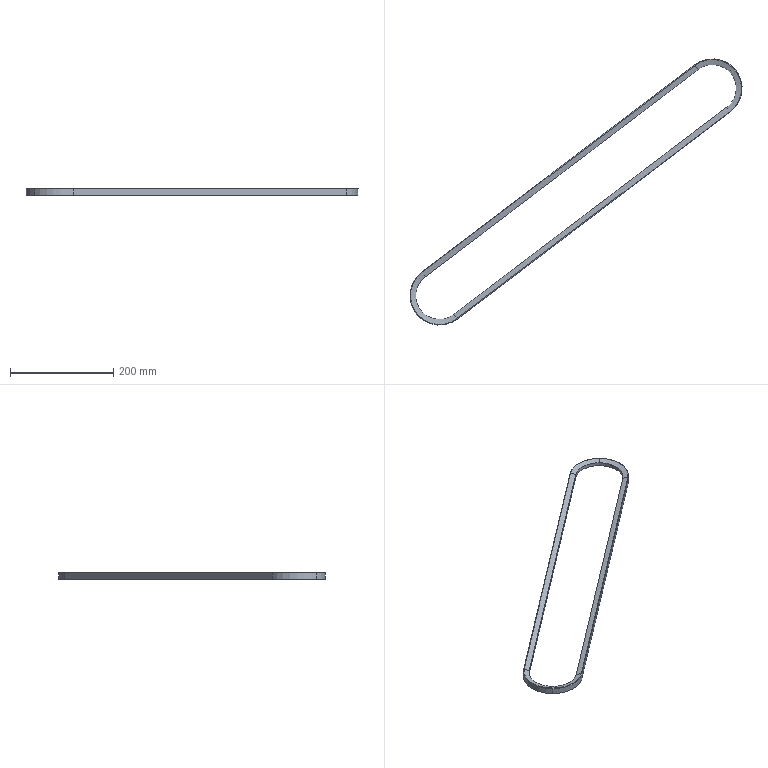Component | SolidWorks | Belt-1 | 1 solid | 30 faces | box 643.7 x 516.05 x 13.2 mm | volume 188359 mm3 | cone 12 | plane 12 | cylinder 6 | commonest cylinder face diameters 114 x3 92 x3
STEP:
#1=COLOUR_RGB('',0.7922,0.8196,0.9333);
#2=FILL_AREA_STYLE_COLOUR('',#1);
#3=FILL_AREA_STYLE('',(#2));
#4=SURFACE_STYLE_FILL_AREA(#3);
#5=SURFACE_SIDE_STYLE('',(#4));
#6=SURFACE_STYLE_USAGE(.BOTH.,#5);
#7=PRESENTATION_STYLE_ASSIGNMENT((#6));
#8=CARTESIAN_POINT('',(-11.222,-8.795,-9.154));
#9=VERTEX_POINT('',#8);
#10=CARTESIAN_POINT('',(-14.155,-8.605,-9.154));
#11=VERTEX_POINT('',#10);
#12=CARTESIAN_POINT('',(-12.579,-7.008,-9.154));
#13=DIRECTION('',(0.,0.,-1.));
#14=DIRECTION('',(-0.7024,-0.7117,0.));
#15=AXIS2_PLACEMENT_3D('',#12,#13,#14);
#16=CIRCLE('',#15,2.244);
#17=EDGE_CURVE('',#9,#11,#16,.T.);
#18=ORIENTED_EDGE('',*,*,#17,.T.);
#19=CARTESIAN_POINT('',(-14.155,-8.605,-9.618));
#20=VERTEX_POINT('',#19);
#21=CARTESIAN_POINT('',(-14.155,-8.605,-9.386));
#22=DIRECTION('',(0.,0.,-1.));
#23=VECTOR('',#22,39.37);
#24=LINE('',#21,#23);
#25=EDGE_CURVE('',#11,#20,#24,.T.);
#26=ORIENTED_EDGE('',*,*,#25,.T.);
#27=CARTESIAN_POINT('',(-11.222,-8.795,-9.618));
#28=VERTEX_POINT('',#27);
#29=CARTESIAN_POINT('',(-12.579,-7.008,-9.618));
#30=DIRECTION('',(0.,0.,1.));
#31=DIRECTION('',(-0.7024,-0.7117,0.));
#32=AXIS2_PLACEMENT_3D('',#29,#30,#31);
#33=CIRCLE('',#32,2.244);
#34=EDGE_CURVE('',#20,#28,#33,.T.);
#35=ORIENTED_EDGE('',*,*,#34,.T.);
#36=CARTESIAN_POINT('',(-11.222,-8.795,-9.386));
#37=DIRECTION('',(0.,0.,1.));
#38=VECTOR('',#37,39.37);
#39=LINE('',#36,#38);
#40=EDGE_CURVE('',#28,#9,#39,.T.);
#41=ORIENTED_EDGE('',*,*,#40,.T.);
#42=EDGE_LOOP('',(#18,#26,#35,#41));
#43=FACE_OUTER_BOUND('',#42,.T.);
#44=CARTESIAN_POINT('',(-12.579,-7.008,-9.386));
#45=DIRECTION('',(0.,0.,-1.));
#46=DIRECTION('',(-0.7024,-0.7117,0.));
#47=AXIS2_PLACEMENT_3D('',#44,#45,#46);
#48=CYLINDRICAL_SURFACE('',#47,2.244);
#49=ADVANCED_FACE('',(#43),#48,.T.);
#50=CARTESIAN_POINT('',(-11.245,-8.765,-9.126));
#51=VERTEX_POINT('',#50);
#52=CARTESIAN_POINT('',(-14.129,-8.578,-9.126));
#53=VERTEX_POINT('',#52);
#54=CARTESIAN_POINT('',(-12.579,-7.008,-9.126));
#55=DIRECTION('',(0.,0.,-1.));
#56=DIRECTION('',(-0.7024,-0.7117,0.));
#57=AXIS2_PLACEMENT_3D('',#54,#55,#56);
#58=CIRCLE('',#57,2.206);
#59=EDGE_CURVE('',#51,#53,#58,.T.);
#60=ORIENTED_EDGE('',*,*,#59,.T.);
#61=CARTESIAN_POINT('',(-14.155,-8.605,-9.154));
#62=DIRECTION('',(-0.5647,-0.5721,-0.5948));
#63=VECTOR('',#62,39.37);
#64=LINE('',#61,#63);
#65=EDGE_CURVE('',#53,#11,#64,.T.);
#66=ORIENTED_EDGE('',*,*,#65,.T.);
#67=ORIENTED_EDGE('',*,*,#17,.F.);
#68=CARTESIAN_POINT('',(-11.245,-8.765,-9.126));
#69=DIRECTION('',(-0.486,0.6403,0.5948));
#70=VECTOR('',#69,39.37);
#71=LINE('',#68,#70);
#72=EDGE_CURVE('',#9,#51,#71,.T.);
#73=ORIENTED_EDGE('',*,*,#72,.T.);
#74=EDGE_LOOP('',(#60,#66,#67,#73));
#75=FACE_OUTER_BOUND('',#74,.T.);
#76=CARTESIAN_POINT('',(-12.579,-7.008,-9.154));
#77=DIRECTION('',(0.,0.,-1.));
#78=DIRECTION('',(-0.7024,-0.7117,0.));
#79=AXIS2_PLACEMENT_3D('',#76,#77,#78);
#80=CONICAL_SURFACE('',#79,2.244,0.9338);
#81=ADVANCED_FACE('',(#75),#80,.T.);
#82=CARTESIAN_POINT('',(9.61,7.063,-9.646));
#83=VERTEX_POINT('',#82);
#84=CARTESIAN_POINT('',(9.826,10.391,-9.646));
#85=VERTEX_POINT('',#84);
#86=CARTESIAN_POINT('',(8.276,8.821,-9.646));
#87=DIRECTION('',(0.,0.,1.));
#88=DIRECTION('',(0.7024,0.7117,0.));
#89=AXIS2_PLACEMENT_3D('',#86,#87,#88);
#90=CIRCLE('',#89,2.206);
#91=EDGE_CURVE('',#83,#85,#90,.T.);
#92=ORIENTED_EDGE('',*,*,#91,.T.);
#93=CARTESIAN_POINT('',(9.852,10.418,-9.618));
#94=VERTEX_POINT('',#93);
#95=CARTESIAN_POINT('',(9.852,10.418,-9.618));
#96=DIRECTION('',(0.5647,0.5721,0.5948));
#97=VECTOR('',#96,39.37);
#98=LINE('',#95,#97);
#99=EDGE_CURVE('',#85,#94,#98,.T.);
#100=ORIENTED_EDGE('',*,*,#99,.T.);
#101=CARTESIAN_POINT('',(9.632,7.033,-9.618));
#102=VERTEX_POINT('',#101);
#103=CARTESIAN_POINT('',(8.276,8.821,-9.618));
#104=DIRECTION('',(0.,0.,1.));
#105=DIRECTION('',(-0.7024,-0.7117,0.));
#106=AXIS2_PLACEMENT_3D('',#103,#104,#105);
#107=CIRCLE('',#106,2.244);
#108=EDGE_CURVE('',#102,#94,#107,.T.);
#109=ORIENTED_EDGE('',*,*,#108,.F.);
#110=CARTESIAN_POINT('',(9.632,7.033,-9.618));
#111=DIRECTION('',(-0.486,0.6403,-0.5948));
#112=VECTOR('',#111,39.37);
#113=LINE('',#110,#112);
#114=EDGE_CURVE('',#102,#83,#113,.T.);
#115=ORIENTED_EDGE('',*,*,#114,.T.);
#116=EDGE_LOOP('',(#92,#100,#109,#115));
#117=FACE_OUTER_BOUND('',#116,.T.);
#118=CARTESIAN_POINT('',(8.276,8.821,-9.618));
#119=DIRECTION('',(0.,0.,1.));
#120=DIRECTION('',(0.7024,0.7117,0.));
#121=AXIS2_PLACEMENT_3D('',#118,#119,#120);
#122=CONICAL_SURFACE('',#121,2.244,0.9338);
#123=ADVANCED_FACE('',(#117),#122,.T.);
#124=CARTESIAN_POINT('',(-13.868,-5.736,-9.525));
#125=VERTEX_POINT('',#124);
#126=CARTESIAN_POINT('',(-13.674,-5.565,-9.525));
#127=VERTEX_POINT('',#126);
#128=CARTESIAN_POINT('',(-12.579,-7.008,-9.525));
#129=DIRECTION('',(0.,0.,-1.));
#130=DIRECTION('',(-0.7024,-0.7117,0.));
#131=AXIS2_PLACEMENT_3D('',#128,#129,#130);
#132=CIRCLE('',#131,1.811);
#133=EDGE_CURVE('',#125,#127,#132,.T.);
#134=ORIENTED_EDGE('',*,*,#133,.F.);
#135=CARTESIAN_POINT('',(-14.149,-5.458,-9.646));
#136=VERTEX_POINT('',#135);
#137=CARTESIAN_POINT('',(-14.149,-5.458,-9.646));
#138=DIRECTION('',(-0.6806,0.6717,-0.2924));
#139=VECTOR('',#138,39.37);
#140=LINE('',#137,#139);
#141=EDGE_CURVE('',#125,#136,#140,.T.);
#142=ORIENTED_EDGE('',*,*,#141,.T.);
#143=CARTESIAN_POINT('',(-13.913,-5.25,-9.646));
#144=VERTEX_POINT('',#143);
#145=CARTESIAN_POINT('',(-12.579,-7.008,-9.646));
#146=DIRECTION('',(0.,0.,1.));
#147=DIRECTION('',(0.7024,0.7117,0.));
#148=AXIS2_PLACEMENT_3D('',#145,#146,#147);
#149=CIRCLE('',#148,2.206);
#150=EDGE_CURVE('',#144,#136,#149,.T.);
#151=ORIENTED_EDGE('',*,*,#150,.F.);
#152=CARTESIAN_POINT('',(-13.913,-5.25,-9.646));
#153=DIRECTION('',(0.5782,-0.7617,0.2924));
#154=VECTOR('',#153,39.37);
#155=LINE('',#152,#154);
#156=EDGE_CURVE('',#144,#127,#155,.T.);
#157=ORIENTED_EDGE('',*,*,#156,.T.);
#158=EDGE_LOOP('',(#134,#142,#151,#157));
#159=FACE_OUTER_BOUND('',#158,.T.);
#160=CARTESIAN_POINT('',(-12.579,-7.008,-9.646));
#161=DIRECTION('',(-0.,0.,-1.));
#162=DIRECTION('',(-0.7117,0.7024,0.));
#163=AXIS2_PLACEMENT_3D('',#160,#161,#162);
#164=CONICAL_SURFACE('',#163,2.206,1.274);
#165=ADVANCED_FACE('',(#159),#164,.F.);
#166=CARTESIAN_POINT('',(9.548,10.11,-9.247));
#167=VERTEX_POINT('',#166);
#168=CARTESIAN_POINT('',(7.181,10.263,-9.247));
#169=VERTEX_POINT('',#168);
#170=CARTESIAN_POINT('',(8.276,8.821,-9.247));
#171=DIRECTION('',(0.,0.,1.));
#172=DIRECTION('',(0.7024,0.7117,0.));
#173=AXIS2_PLACEMENT_3D('',#170,#171,#172);
#174=CIRCLE('',#173,1.811);
#175=EDGE_CURVE('',#167,#169,#174,.T.);
#176=ORIENTED_EDGE('',*,*,#175,.F.);
#177=CARTESIAN_POINT('',(9.826,10.391,-9.126));
#178=VERTEX_POINT('',#177);
#179=CARTESIAN_POINT('',(9.826,10.391,-9.126));
#180=DIRECTION('',(0.6717,0.6806,0.2924));
#181=VECTOR('',#180,39.37);
#182=LINE('',#179,#181);
#183=EDGE_CURVE('',#167,#178,#182,.T.);
#184=ORIENTED_EDGE('',*,*,#183,.T.);
#185=CARTESIAN_POINT('',(6.942,10.578,-9.126));
#186=VERTEX_POINT('',#185);
#187=CARTESIAN_POINT('',(8.276,8.821,-9.126));
#188=DIRECTION('',(0.,0.,-1.));
#189=DIRECTION('',(-0.7024,-0.7117,0.));
#190=AXIS2_PLACEMENT_3D('',#187,#188,#189);
#191=CIRCLE('',#190,2.206);
#192=EDGE_CURVE('',#186,#178,#191,.T.);
#193=ORIENTED_EDGE('',*,*,#192,.F.);
#194=CARTESIAN_POINT('',(6.942,10.578,-9.126));
#195=DIRECTION('',(0.5782,-0.7617,-0.2924));
#196=VECTOR('',#195,39.37);
#197=LINE('',#194,#196);
#198=EDGE_CURVE('',#186,#169,#197,.T.);
#199=ORIENTED_EDGE('',*,*,#198,.T.);
#200=EDGE_LOOP('',(#176,#184,#193,#199));
#201=FACE_OUTER_BOUND('',#200,.T.);
#202=CARTESIAN_POINT('',(8.276,8.821,-9.126));
#203=DIRECTION('',(0.,0.,1.));
#204=DIRECTION('',(0.7024,0.7117,0.));
#205=AXIS2_PLACEMENT_3D('',#202,#203,#204);
#206=CONICAL_SURFACE('',#205,2.206,1.274);
#207=ADVANCED_FACE('',(#201),#206,.F.);
#208=CARTESIAN_POINT('',(-13.674,-5.565,-9.247));
#209=VERTEX_POINT('',#208);
#210=CARTESIAN_POINT('',(-13.851,-8.297,-9.247));
#211=VERTEX_POINT('',#210);
#212=CARTESIAN_POINT('',(-12.579,-7.008,-9.247));
#213=DIRECTION('',(0.,0.,1.));
#214=DIRECTION('',(0.7024,0.7117,0.));
#215=AXIS2_PLACEMENT_3D('',#212,#213,#214);
#216=CIRCLE('',#215,1.811);
#217=EDGE_CURVE('',#209,#211,#216,.T.);
#218=ORIENTED_EDGE('',*,*,#217,.T.);
#219=CARTESIAN_POINT('',(-13.851,-8.297,-9.525));
#220=VERTEX_POINT('',#219);
#221=CARTESIAN_POINT('',(-13.851,-8.297,-9.386));
#222=DIRECTION('',(0.,0.,-1.));
#223=VECTOR('',#222,39.37);
#224=LINE('',#221,#223);
#225=EDGE_CURVE('',#211,#220,#224,.T.);
#226=ORIENTED_EDGE('',*,*,#225,.T.);
#227=CARTESIAN_POINT('',(-12.579,-7.008,-9.525));
#228=DIRECTION('',(0.,0.,-1.));
#229=DIRECTION('',(-0.7024,-0.7117,0.));
#230=AXIS2_PLACEMENT_3D('',#227,#228,#229);
#231=CIRCLE('',#230,1.811);
#232=EDGE_CURVE('',#220,#125,#231,.T.);
#233=ORIENTED_EDGE('',*,*,#232,.T.);
#234=ORIENTED_EDGE('',*,*,#133,.T.);
#235=CARTESIAN_POINT('',(-13.674,-5.565,-9.525));
#236=DIRECTION('',(0.,0.,1.));
#237=VECTOR('',#236,39.37);
#238=LINE('',#235,#237);
#239=EDGE_CURVE('',#127,#209,#238,.T.);
#240=ORIENTED_EDGE('',*,*,#239,.T.);
#241=EDGE_LOOP('',(#218,#226,#233,#234,#240));
#242=FACE_OUTER_BOUND('',#241,.T.);
#243=CARTESIAN_POINT('',(-12.579,-7.008,-9.386));
#244=DIRECTION('',(0.,0.,-1.));
#245=DIRECTION('',(-0.7024,-0.7117,0.));
#246=AXIS2_PLACEMENT_3D('',#243,#244,#245);
#247=CYLINDRICAL_SURFACE('',#246,1.811);
#248=ADVANCED_FACE('',(#242),#247,.F.);
#249=CARTESIAN_POINT('',(6.919,10.608,-9.154));
#250=VERTEX_POINT('',#249);
#251=CARTESIAN_POINT('',(-13.935,-5.22,-9.154));
#252=VERTEX_POINT('',#251);
#253=CARTESIAN_POINT('',(-13.935,-5.22,-9.154));
#254=DIRECTION('',(-0.7965,-0.6046,0.));
#255=VECTOR('',#254,39.37);
#256=LINE('',#253,#255);
#257=EDGE_CURVE('',#250,#252,#256,.T.);
#258=ORIENTED_EDGE('',*,*,#257,.F.);
#259=CARTESIAN_POINT('',(6.919,10.608,-9.618));
#260=VERTEX_POINT('',#259);
#261=CARTESIAN_POINT('',(6.919,10.608,-9.618));
#262=DIRECTION('',(0.,0.,1.));
#263=VECTOR('',#262,39.37);
#264=LINE('',#261,#263);
#265=EDGE_CURVE('',#260,#250,#264,.T.);
#266=ORIENTED_EDGE('',*,*,#265,.F.);
#267=CARTESIAN_POINT('',(-13.935,-5.22,-9.618));
#268=VERTEX_POINT('',#267);
#269=CARTESIAN_POINT('',(-13.935,-5.22,-9.618));
#270=DIRECTION('',(0.7965,0.6046,0.));
#271=VECTOR('',#270,39.37);
#272=LINE('',#269,#271);
#273=EDGE_CURVE('',#268,#260,#272,.T.);
#274=ORIENTED_EDGE('',*,*,#273,.F.);
#275=CARTESIAN_POINT('',(-13.935,-5.22,-9.618));
#276=DIRECTION('',(0.,0.,-1.));
#277=VECTOR('',#276,39.37);
#278=LINE('',#275,#277);
#279=EDGE_CURVE('',#252,#268,#278,.T.);
#280=ORIENTED_EDGE('',*,*,#279,.F.);
#281=EDGE_LOOP('',(#258,#266,#274,#280));
#282=FACE_OUTER_BOUND('',#281,.T.);
#283=CARTESIAN_POINT('',(-13.935,-5.22,-9.618));
#284=DIRECTION('',(0.6046,-0.7965,0.));
#285=DIRECTION('',(0.7965,0.6046,0.));
#286=AXIS2_PLACEMENT_3D('',#283,#284,#285);
#287=PLANE('',#286);
#288=ADVANCED_FACE('',(#282),#287,.F.);
#289=ORIENTED_EDGE('',*,*,#25,.F.);
#290=CARTESIAN_POINT('',(-12.579,-7.008,-9.154));
#291=DIRECTION('',(0.,0.,-1.));
#292=DIRECTION('',(-0.7024,-0.7117,0.));
#293=AXIS2_PLACEMENT_3D('',#290,#291,#292);
#294=CIRCLE('',#293,2.244);
#295=EDGE_CURVE('',#11,#252,#294,.T.);
#296=ORIENTED_EDGE('',*,*,#295,.T.);
#297=ORIENTED_EDGE('',*,*,#279,.T.);
#298=CARTESIAN_POINT('',(-12.579,-7.008,-9.618));
#299=DIRECTION('',(0.,0.,1.));
#300=DIRECTION('',(-0.7024,-0.7117,0.));
#301=AXIS2_PLACEMENT_3D('',#298,#299,#300);
#302=CIRCLE('',#301,2.244);
#303=EDGE_CURVE('',#268,#20,#302,.T.);
#304=ORIENTED_EDGE('',*,*,#303,.T.);
#305=EDGE_LOOP('',(#289,#296,#297,#304));
#306=FACE_OUTER_BOUND('',#305,.T.);
#307=CARTESIAN_POINT('',(-12.579,-7.008,-9.386));
#308=DIRECTION('',(0.,0.,-1.));
#309=DIRECTION('',(-0.7024,-0.7117,0.));
#310=AXIS2_PLACEMENT_3D('',#307,#308,#309);
#311=CYLINDRICAL_SURFACE('',#310,2.244);
#312=ADVANCED_FACE('',(#306),#311,.T.);
#313=CARTESIAN_POINT('',(-13.913,-5.25,-9.126));
#314=VERTEX_POINT('',#313);
#315=CARTESIAN_POINT('',(6.942,10.578,-9.126));
#316=DIRECTION('',(-0.7965,-0.6046,0.));
#317=VECTOR('',#316,39.37);
#318=LINE('',#315,#317);
#319=EDGE_CURVE('',#186,#314,#318,.T.);
#320=ORIENTED_EDGE('',*,*,#319,.F.);
#321=CARTESIAN_POINT('',(6.942,10.578,-9.126));
#322=DIRECTION('',(0.486,-0.6403,0.5948));
#323=VECTOR('',#322,39.37);
#324=LINE('',#321,#323);
#325=EDGE_CURVE('',#250,#186,#324,.T.);
#326=ORIENTED_EDGE('',*,*,#325,.F.);
#327=ORIENTED_EDGE('',*,*,#257,.T.);
#328=CARTESIAN_POINT('',(-13.913,-5.25,-9.126));
#329=DIRECTION('',(-0.486,0.6403,-0.5948));
#330=VECTOR('',#329,39.37);
#331=LINE('',#328,#330);
#332=EDGE_CURVE('',#314,#252,#331,.T.);
#333=ORIENTED_EDGE('',*,*,#332,.F.);
#334=EDGE_LOOP('',(#320,#326,#327,#333));
#335=FACE_OUTER_BOUND('',#334,.T.);
#336=CARTESIAN_POINT('',(-13.935,-5.22,-9.154));
#337=DIRECTION('',(0.3596,-0.4738,-0.8039));
#338=DIRECTION('',(-0.5742,0.5667,-0.5909));
#339=AXIS2_PLACEMENT_3D('',#336,#337,#338);
#340=PLANE('',#339);
#341=ADVANCED_FACE('',(#335),#340,.F.);
#342=CARTESIAN_POINT('',(9.632,7.033,-9.154));
#343=VERTEX_POINT('',#342);
#344=CARTESIAN_POINT('',(8.276,8.821,-9.154));
#345=DIRECTION('',(0.,0.,-1.));
#346=DIRECTION('',(-0.7024,-0.7117,0.));
#347=AXIS2_PLACEMENT_3D('',#344,#345,#346);
#348=CIRCLE('',#347,2.244);
#349=EDGE_CURVE('',#250,#343,#348,.T.);
#350=ORIENTED_EDGE('',*,*,#349,.T.);
#351=CARTESIAN_POINT('',(9.632,7.033,-9.386));
#352=DIRECTION('',(0.,0.,-1.));
#353=VECTOR('',#352,39.37);
#354=LINE('',#351,#353);
#355=EDGE_CURVE('',#343,#102,#354,.T.);
#356=ORIENTED_EDGE('',*,*,#355,.T.);
#357=ORIENTED_EDGE('',*,*,#108,.T.);
#358=CARTESIAN_POINT('',(8.276,8.821,-9.618));
#359=DIRECTION('',(0.,0.,1.));
#360=DIRECTION('',(-0.7024,-0.7117,0.));
#361=AXIS2_PLACEMENT_3D('',#358,#359,#360);
#362=CIRCLE('',#361,2.244);
#363=EDGE_CURVE('',#94,#260,#362,.T.);
#364=ORIENTED_EDGE('',*,*,#363,.T.);
#365=ORIENTED_EDGE('',*,*,#265,.T.);
#366=EDGE_LOOP('',(#350,#356,#357,#364,#365));
#367=FACE_OUTER_BOUND('',#366,.T.);
#368=CARTESIAN_POINT('',(8.276,8.821,-9.386));
#369=DIRECTION('',(0.,0.,-1.));
#370=DIRECTION('',(-0.7024,-0.7117,0.));
#371=AXIS2_PLACEMENT_3D('',#368,#369,#370);
#372=CYLINDRICAL_SURFACE('',#371,2.244);
#373=ADVANCED_FACE('',(#367),#372,.T.);
#374=ORIENTED_EDGE('',*,*,#273,.T.);
#375=CARTESIAN_POINT('',(6.942,10.578,-9.646));
#376=VERTEX_POINT('',#375);
#377=CARTESIAN_POINT('',(6.942,10.578,-9.646));
#378=DIRECTION('',(-0.486,0.6403,0.5948));
#379=VECTOR('',#378,39.37);
#380=LINE('',#377,#379);
#381=EDGE_CURVE('',#376,#260,#380,.T.);
#382=ORIENTED_EDGE('',*,*,#381,.F.);
#383=CARTESIAN_POINT('',(-13.913,-5.25,-9.646));
#384=DIRECTION('',(0.7965,0.6046,0.));
#385=VECTOR('',#384,39.37);
#386=LINE('',#383,#385);
#387=EDGE_CURVE('',#144,#376,#386,.T.);
#388=ORIENTED_EDGE('',*,*,#387,.F.);
#389=CARTESIAN_POINT('',(-13.935,-5.22,-9.618));
#390=DIRECTION('',(0.486,-0.6403,-0.5948));
#391=VECTOR('',#390,39.37);
#392=LINE('',#389,#391);
#393=EDGE_CURVE('',#268,#144,#392,.T.);
#394=ORIENTED_EDGE('',*,*,#393,.F.);
#395=EDGE_LOOP('',(#374,#382,#388,#394));
#396=FACE_OUTER_BOUND('',#395,.T.);
#397=CARTESIAN_POINT('',(-13.913,-5.25,-9.646));
#398=DIRECTION('',(0.3596,-0.4738,0.8039));
#399=DIRECTION('',(0.5742,-0.5667,-0.5909));
#400=AXIS2_PLACEMENT_3D('',#397,#398,#399);
#401=PLANE('',#400);
#402=ADVANCED_FACE('',(#396),#401,.F.);
#403=ORIENTED_EDGE('',*,*,#393,.T.);
#404=ORIENTED_EDGE('',*,*,#150,.T.);
#405=CARTESIAN_POINT('',(-11.245,-8.765,-9.646));
#406=VERTEX_POINT('',#405);
#407=CARTESIAN_POINT('',(-12.579,-7.008,-9.646));
#408=DIRECTION('',(0.,0.,1.));
#409=DIRECTION('',(0.7024,0.7117,0.));
#410=AXIS2_PLACEMENT_3D('',#407,#408,#409);
#411=CIRCLE('',#410,2.206);
#412=EDGE_CURVE('',#136,#406,#411,.T.);
#413=ORIENTED_EDGE('',*,*,#412,.T.);
#414=CARTESIAN_POINT('',(-11.245,-8.765,-9.646));
#415=DIRECTION('',(0.486,-0.6403,0.5948));
#416=VECTOR('',#415,39.37);
#417=LINE('',#414,#416);
#418=EDGE_CURVE('',#406,#28,#417,.T.);
#419=ORIENTED_EDGE('',*,*,#418,.T.);
#420=ORIENTED_EDGE('',*,*,#34,.F.);
#421=ORIENTED_EDGE('',*,*,#303,.F.);
#422=EDGE_LOOP('',(#403,#404,#413,#419,#420,#421));
#423=FACE_OUTER_BOUND('',#422,.T.);
#424=CARTESIAN_POINT('',(-12.579,-7.008,-9.618));
#425=DIRECTION('',(0.,0.,1.));
#426=DIRECTION('',(0.7024,0.7117,0.));
#427=AXIS2_PLACEMENT_3D('',#424,#425,#426);
#428=CONICAL_SURFACE('',#427,2.244,0.9338);
#429=ADVANCED_FACE('',(#423),#428,.T.);
#430=ORIENTED_EDGE('',*,*,#65,.F.);
#431=CARTESIAN_POINT('',(-12.579,-7.008,-9.126));
#432=DIRECTION('',(0.,0.,-1.));
#433=DIRECTION('',(-0.7024,-0.7117,0.));
#434=AXIS2_PLACEMENT_3D('',#431,#432,#433);
#435=CIRCLE('',#434,2.206);
#436=EDGE_CURVE('',#53,#314,#435,.T.);
#437=ORIENTED_EDGE('',*,*,#436,.T.);
#438=ORIENTED_EDGE('',*,*,#332,.T.);
#439=ORIENTED_EDGE('',*,*,#295,.F.);
#440=EDGE_LOOP('',(#430,#437,#438,#439));
#441=FACE_OUTER_BOUND('',#440,.T.);
#442=CARTESIAN_POINT('',(-12.579,-7.008,-9.154));
#443=DIRECTION('',(0.,0.,-1.));
#444=DIRECTION('',(-0.7024,-0.7117,0.));
#445=AXIS2_PLACEMENT_3D('',#442,#443,#444);
#446=CONICAL_SURFACE('',#445,2.244,0.9338);
#447=ADVANCED_FACE('',(#441),#446,.T.);
#448=CARTESIAN_POINT('',(7.181,10.263,-9.247));
#449=DIRECTION('',(-0.7965,-0.6046,-0.));
#450=VECTOR('',#449,39.37);
#451=LINE('',#448,#450);
#452=EDGE_CURVE('',#169,#209,#451,.T.);
#453=ORIENTED_EDGE('',*,*,#452,.F.);
#454=ORIENTED_EDGE('',*,*,#198,.F.);
#455=ORIENTED_EDGE('',*,*,#319,.T.);
#456=CARTESIAN_POINT('',(-13.674,-5.565,-9.247));
#457=DIRECTION('',(-0.5782,0.7617,0.2924));
#458=VECTOR('',#457,39.37);
#459=LINE('',#456,#458);
#460=EDGE_CURVE('',#209,#314,#459,.T.);
#461=ORIENTED_EDGE('',*,*,#460,.F.);
#462=EDGE_LOOP('',(#453,#454,#455,#461));
#463=FACE_OUTER_BOUND('',#462,.T.);
#464=CARTESIAN_POINT('',(-13.913,-5.25,-9.126));
#465=DIRECTION('',(-0.1768,0.2329,-0.9563));
#466=DIRECTION('',(-0.6812,0.6723,0.2896));
#467=AXIS2_PLACEMENT_3D('',#464,#465,#466);
#468=PLANE('',#467);
#469=ADVANCED_FACE('',(#463),#468,.F.);
#470=ORIENTED_EDGE('',*,*,#99,.F.);
#471=CARTESIAN_POINT('',(8.276,8.821,-9.646));
#472=DIRECTION('',(0.,0.,1.));
#473=DIRECTION('',(0.7024,0.7117,0.));
#474=AXIS2_PLACEMENT_3D('',#471,#472,#473);
#475=CIRCLE('',#474,2.206);
#476=EDGE_CURVE('',#85,#376,#475,.T.);
#477=ORIENTED_EDGE('',*,*,#476,.T.);
#478=ORIENTED_EDGE('',*,*,#381,.T.);
#479=ORIENTED_EDGE('',*,*,#363,.F.);
#480=EDGE_LOOP('',(#470,#477,#478,#479));
#481=FACE_OUTER_BOUND('',#480,.T.);
#482=CARTESIAN_POINT('',(8.276,8.821,-9.618));
#483=DIRECTION('',(0.,0.,1.));
#484=DIRECTION('',(0.7024,0.7117,0.));
#485=AXIS2_PLACEMENT_3D('',#482,#483,#484);
#486=CONICAL_SURFACE('',#485,2.244,0.9338);
#487=ADVANCED_FACE('',(#481),#486,.T.);
#488=ORIENTED_EDGE('',*,*,#192,.T.);
#489=CARTESIAN_POINT('',(9.61,7.063,-9.126));
#490=VERTEX_POINT('',#489);
#491=CARTESIAN_POINT('',(8.276,8.821,-9.126));
#492=DIRECTION('',(0.,0.,-1.));
#493=DIRECTION('',(-0.7024,-0.7117,0.));
#494=AXIS2_PLACEMENT_3D('',#491,#492,#493);
#495=CIRCLE('',#494,2.206);
#496=EDGE_CURVE('',#178,#490,#495,.T.);
#497=ORIENTED_EDGE('',*,*,#496,.T.);
#498=CARTESIAN_POINT('',(9.61,7.063,-9.126));
#499=DIRECTION('',(0.486,-0.6403,-0.5948));
#500=VECTOR('',#499,39.37);
#501=LINE('',#498,#500);
#502=EDGE_CURVE('',#490,#343,#501,.T.);
#503=ORIENTED_EDGE('',*,*,#502,.T.);
#504=ORIENTED_EDGE('',*,*,#349,.F.);
#505=ORIENTED_EDGE('',*,*,#325,.T.);
#506=EDGE_LOOP('',(#488,#497,#503,#504,#505));
#507=FACE_OUTER_BOUND('',#506,.T.);
#508=CARTESIAN_POINT('',(8.276,8.821,-9.154));
#509=DIRECTION('',(0.,0.,-1.));
#510=DIRECTION('',(-0.7024,-0.7117,0.));
#511=AXIS2_PLACEMENT_3D('',#508,#509,#510);
#512=CONICAL_SURFACE('',#511,2.244,0.9338);
#513=ADVANCED_FACE('',(#507),#512,.T.);
#514=ORIENTED_EDGE('',*,*,#387,.T.);
#515=CARTESIAN_POINT('',(7.181,10.263,-9.525));
#516=VERTEX_POINT('',#515);
#517=CARTESIAN_POINT('',(7.181,10.263,-9.525));
#518=DIRECTION('',(-0.5782,0.7617,-0.2924));
#519=VECTOR('',#518,39.37);
#520=LINE('',#517,#519);
#521=EDGE_CURVE('',#516,#376,#520,.T.);
#522=ORIENTED_EDGE('',*,*,#521,.F.);
#523=CARTESIAN_POINT('',(-13.674,-5.565,-9.525));
#524=DIRECTION('',(0.7965,0.6046,0.));
#525=VECTOR('',#524,39.37);
#526=LINE('',#523,#525);
#527=EDGE_CURVE('',#127,#516,#526,.T.);
#528=ORIENTED_EDGE('',*,*,#527,.F.);
#529=ORIENTED_EDGE('',*,*,#156,.F.);
#530=EDGE_LOOP('',(#514,#522,#528,#529));
#531=FACE_OUTER_BOUND('',#530,.T.);
#532=CARTESIAN_POINT('',(-13.674,-5.565,-9.525));
#533=DIRECTION('',(-0.1768,0.2329,0.9563));
#534=DIRECTION('',(0.6812,-0.6723,0.2896));
#535=AXIS2_PLACEMENT_3D('',#532,#533,#534);
#536=PLANE('',#535);
#537=ADVANCED_FACE('',(#531),#536,.F.);
#538=ORIENTED_EDGE('',*,*,#141,.F.);
#539=ORIENTED_EDGE('',*,*,#232,.F.);
#540=CARTESIAN_POINT('',(-11.484,-8.45,-9.525));
#541=VERTEX_POINT('',#540);
#542=CARTESIAN_POINT('',(-12.579,-7.008,-9.525));
#543=DIRECTION('',(0.,0.,-1.));
#544=DIRECTION('',(-0.7024,-0.7117,0.));
#545=AXIS2_PLACEMENT_3D('',#542,#543,#544);
#546=CIRCLE('',#545,1.811);
#547=EDGE_CURVE('',#541,#220,#546,.T.);
#548=ORIENTED_EDGE('',*,*,#547,.F.);
#549=CARTESIAN_POINT('',(-11.245,-8.765,-9.646));
#550=DIRECTION('',(-0.5782,0.7617,0.2924));
#551=VECTOR('',#550,39.37);
#552=LINE('',#549,#551);
#553=EDGE_CURVE('',#406,#541,#552,.T.);
#554=ORIENTED_EDGE('',*,*,#553,.F.);
#555=ORIENTED_EDGE('',*,*,#412,.F.);
#556=EDGE_LOOP('',(#538,#539,#548,#554,#555));
#557=FACE_OUTER_BOUND('',#556,.T.);
#558=CARTESIAN_POINT('',(-12.579,-7.008,-9.646));
#559=DIRECTION('',(-0.,0.,-1.));
#560=DIRECTION('',(-0.7117,0.7024,0.));
#561=AXIS2_PLACEMENT_3D('',#558,#559,#560);
#562=CONICAL_SURFACE('',#561,2.206,1.274);
#563=ADVANCED_FACE('',(#557),#562,.F.);
#564=ORIENTED_EDGE('',*,*,#217,.F.);
#565=ORIENTED_EDGE('',*,*,#460,.T.);
#566=ORIENTED_EDGE('',*,*,#436,.F.);
#567=ORIENTED_EDGE('',*,*,#59,.F.);
#568=CARTESIAN_POINT('',(-11.484,-8.45,-9.247));
#569=VERTEX_POINT('',#568);
#570=CARTESIAN_POINT('',(-11.484,-8.45,-9.247));
#571=DIRECTION('',(0.5782,-0.7617,0.2924));
#572=VECTOR('',#571,39.37);
#573=LINE('',#570,#572);
#574=EDGE_CURVE('',#569,#51,#573,.T.);
#575=ORIENTED_EDGE('',*,*,#574,.F.);
#576=CARTESIAN_POINT('',(-12.579,-7.008,-9.247));
#577=DIRECTION('',(0.,0.,1.));
#578=DIRECTION('',(0.7024,0.7117,0.));
#579=AXIS2_PLACEMENT_3D('',#576,#577,#578);
#580=CIRCLE('',#579,1.811);
#581=EDGE_CURVE('',#211,#569,#580,.T.);
#582=ORIENTED_EDGE('',*,*,#581,.F.);
#583=EDGE_LOOP('',(#564,#565,#566,#567,#575,#582));
#584=FACE_OUTER_BOUND('',#583,.T.);
#585=CARTESIAN_POINT('',(-12.579,-7.008,-9.126));
#586=DIRECTION('',(0.,0.,1.));
#587=DIRECTION('',(0.7024,0.7117,0.));
#588=AXIS2_PLACEMENT_3D('',#585,#586,#587);
#589=CONICAL_SURFACE('',#588,2.206,1.274);
#590=ADVANCED_FACE('',(#584),#589,.F.);
#591=CARTESIAN_POINT('',(9.632,7.033,-9.154));
#592=DIRECTION('',(0.7965,0.6046,0.));
#593=VECTOR('',#592,39.37);
#594=LINE('',#591,#593);
#595=EDGE_CURVE('',#9,#343,#594,.T.);
#596=ORIENTED_EDGE('',*,*,#595,.F.);
#597=ORIENTED_EDGE('',*,*,#40,.F.);
#598=CARTESIAN_POINT('',(9.632,7.033,-9.618));
#599=DIRECTION('',(-0.7965,-0.6046,0.));
#600=VECTOR('',#599,39.37);
#601=LINE('',#598,#600);
#602=EDGE_CURVE('',#102,#28,#601,.T.);
#603=ORIENTED_EDGE('',*,*,#602,.F.);
#604=ORIENTED_EDGE('',*,*,#355,.F.);
#605=EDGE_LOOP('',(#596,#597,#603,#604));
#606=FACE_OUTER_BOUND('',#605,.T.);
#607=CARTESIAN_POINT('',(9.632,7.033,-9.618));
#608=DIRECTION('',(-0.6046,0.7965,0.));
#609=DIRECTION('',(-0.7965,-0.6046,0.));
#610=AXIS2_PLACEMENT_3D('',#607,#608,#609);
#611=PLANE('',#610);
#612=ADVANCED_FACE('',(#606),#611,.F.);
#613=ORIENTED_EDGE('',*,*,#527,.T.);
#614=CARTESIAN_POINT('',(7.181,10.263,-9.525));
#615=DIRECTION('',(0.,0.,-1.));
#616=VECTOR('',#615,39.37);
#617=LINE('',#614,#616);
#618=EDGE_CURVE('',#169,#516,#617,.T.);
#619=ORIENTED_EDGE('',*,*,#618,.F.);
#620=ORIENTED_EDGE('',*,*,#452,.T.);
#621=ORIENTED_EDGE('',*,*,#239,.F.);
#622=EDGE_LOOP('',(#613,#619,#620,#621));
#623=FACE_OUTER_BOUND('',#622,.T.);
#624=CARTESIAN_POINT('',(-13.674,-5.565,-9.525));
#625=DIRECTION('',(-0.6046,0.7965,0.));
#626=DIRECTION('',(-0.7965,-0.6046,0.));
#627=AXIS2_PLACEMENT_3D('',#624,#625,#626);
#628=PLANE('',#627);
#629=ADVANCED_FACE('',(#623),#628,.F.);
#630=ORIENTED_EDGE('',*,*,#183,.F.);
#631=CARTESIAN_POINT('',(9.371,7.378,-9.247));
#632=VERTEX_POINT('',#631);
#633=CARTESIAN_POINT('',(8.276,8.821,-9.247));
#634=DIRECTION('',(0.,0.,1.));
#635=DIRECTION('',(0.7024,0.7117,0.));
#636=AXIS2_PLACEMENT_3D('',#633,#634,#635);
#637=CIRCLE('',#636,1.811);
#638=EDGE_CURVE('',#632,#167,#637,.T.);
#639=ORIENTED_EDGE('',*,*,#638,.F.);
#640=CARTESIAN_POINT('',(9.371,7.378,-9.247));
#641=DIRECTION('',(0.5782,-0.7617,0.2924));
#642=VECTOR('',#641,39.37);
#643=LINE('',#640,#642);
#644=EDGE_CURVE('',#632,#490,#643,.T.);
#645=ORIENTED_EDGE('',*,*,#644,.T.);
#646=ORIENTED_EDGE('',*,*,#496,.F.);
#647=EDGE_LOOP('',(#630,#639,#645,#646));
#648=FACE_OUTER_BOUND('',#647,.T.);
#649=CARTESIAN_POINT('',(8.276,8.821,-9.126));
#650=DIRECTION('',(0.,0.,1.));
#651=DIRECTION('',(0.7024,0.7117,0.));
#652=AXIS2_PLACEMENT_3D('',#649,#650,#651);
#653=CONICAL_SURFACE('',#652,2.206,1.274);
#654=ADVANCED_FACE('',(#648),#653,.F.);
#655=ORIENTED_EDGE('',*,*,#91,.F.);
#656=CARTESIAN_POINT('',(9.371,7.378,-9.525));
#657=VERTEX_POINT('',#656);
#658=CARTESIAN_POINT('',(9.61,7.063,-9.646));
#659=DIRECTION('',(-0.5782,0.7617,0.2924));
#660=VECTOR('',#659,39.37);
#661=LINE('',#658,#660);
#662=EDGE_CURVE('',#83,#657,#661,.T.);
#663=ORIENTED_EDGE('',*,*,#662,.T.);
#664=CARTESIAN_POINT('',(8.276,8.821,-9.525));
#665=DIRECTION('',(0.,0.,-1.));
#666=DIRECTION('',(-0.7024,-0.7117,0.));
#667=AXIS2_PLACEMENT_3D('',#664,#665,#666);
#668=CIRCLE('',#667,1.811);
#669=EDGE_CURVE('',#516,#657,#668,.T.);
#670=ORIENTED_EDGE('',*,*,#669,.F.);
#671=ORIENTED_EDGE('',*,*,#521,.T.);
#672=ORIENTED_EDGE('',*,*,#476,.F.);
#673=EDGE_LOOP('',(#655,#663,#670,#671,#672));
#674=FACE_OUTER_BOUND('',#673,.T.);
#675=CARTESIAN_POINT('',(8.276,8.821,-9.646));
#676=DIRECTION('',(0.,0.,-1.));
#677=DIRECTION('',(-0.7024,-0.7117,0.));
#678=AXIS2_PLACEMENT_3D('',#675,#676,#677);
#679=CONICAL_SURFACE('',#678,2.206,1.274);
#680=ADVANCED_FACE('',(#674),#679,.F.);
#681=ORIENTED_EDGE('',*,*,#225,.F.);
#682=ORIENTED_EDGE('',*,*,#581,.T.);
#683=CARTESIAN_POINT('',(-11.484,-8.45,-9.386));
#684=DIRECTION('',(0.,0.,1.));
#685=VECTOR('',#684,39.37);
#686=LINE('',#683,#685);
#687=EDGE_CURVE('',#541,#569,#686,.T.);
#688=ORIENTED_EDGE('',*,*,#687,.F.);
#689=ORIENTED_EDGE('',*,*,#547,.T.);
#690=EDGE_LOOP('',(#681,#682,#688,#689));
#691=FACE_OUTER_BOUND('',#690,.T.);
#692=CARTESIAN_POINT('',(-12.579,-7.008,-9.386));
#693=DIRECTION('',(0.,0.,-1.));
#694=DIRECTION('',(-0.7024,-0.7117,0.));
#695=AXIS2_PLACEMENT_3D('',#692,#693,#694);
#696=CYLINDRICAL_SURFACE('',#695,1.811);
#697=ADVANCED_FACE('',(#691),#696,.F.);
#698=CARTESIAN_POINT('',(-11.245,-8.765,-9.646));
#699=DIRECTION('',(0.7965,0.6046,-0.));
#700=VECTOR('',#699,39.37);
#701=LINE('',#698,#700);
#702=EDGE_CURVE('',#406,#83,#701,.T.);
#703=ORIENTED_EDGE('',*,*,#702,.F.);
#704=ORIENTED_EDGE('',*,*,#553,.T.);
#705=CARTESIAN_POINT('',(9.371,7.378,-9.525));
#706=DIRECTION('',(-0.7965,-0.6046,0.));
#707=VECTOR('',#706,39.37);
#708=LINE('',#705,#707);
#709=EDGE_CURVE('',#657,#541,#708,.T.);
#710=ORIENTED_EDGE('',*,*,#709,.F.);
#711=ORIENTED_EDGE('',*,*,#662,.F.);
#712=EDGE_LOOP('',(#703,#704,#710,#711));
#713=FACE_OUTER_BOUND('',#712,.T.);
#714=CARTESIAN_POINT('',(9.371,7.378,-9.525));
#715=DIRECTION('',(0.1768,-0.2329,0.9563));
#716=DIRECTION('',(0.6812,-0.6723,-0.2896));
#717=AXIS2_PLACEMENT_3D('',#714,#715,#716);
#718=PLANE('',#717);
#719=ADVANCED_FACE('',(#713),#718,.F.);
#720=CARTESIAN_POINT('',(-11.484,-8.45,-9.247));
#721=DIRECTION('',(0.7965,0.6046,-0.));
#722=VECTOR('',#721,39.37);
#723=LINE('',#720,#722);
#724=EDGE_CURVE('',#569,#632,#723,.T.);
#725=ORIENTED_EDGE('',*,*,#724,.F.);
#726=ORIENTED_EDGE('',*,*,#574,.T.);
#727=CARTESIAN_POINT('',(9.61,7.063,-9.126));
#728=DIRECTION('',(-0.7965,-0.6046,0.));
#729=VECTOR('',#728,39.37);
#730=LINE('',#727,#729);
#731=EDGE_CURVE('',#490,#51,#730,.T.);
#732=ORIENTED_EDGE('',*,*,#731,.F.);
#733=ORIENTED_EDGE('',*,*,#644,.F.);
#734=EDGE_LOOP('',(#725,#726,#732,#733));
#735=FACE_OUTER_BOUND('',#734,.T.);
#736=CARTESIAN_POINT('',(9.61,7.063,-9.126));
#737=DIRECTION('',(0.1768,-0.2329,-0.9563));
#738=DIRECTION('',(-0.6812,0.6723,-0.2896));
#739=AXIS2_PLACEMENT_3D('',#736,#737,#738);
#740=PLANE('',#739);
#741=ADVANCED_FACE('',(#735),#740,.F.);
#742=ORIENTED_EDGE('',*,*,#731,.T.);
#743=ORIENTED_EDGE('',*,*,#72,.F.);
#744=ORIENTED_EDGE('',*,*,#595,.T.);
#745=ORIENTED_EDGE('',*,*,#502,.F.);
#746=EDGE_LOOP('',(#742,#743,#744,#745));
#747=FACE_OUTER_BOUND('',#746,.T.);
#748=CARTESIAN_POINT('',(9.632,7.033,-9.154));
#749=DIRECTION('',(-0.3596,0.4738,-0.8039));
#750=DIRECTION('',(-0.5742,0.5667,0.5909));
#751=AXIS2_PLACEMENT_3D('',#748,#749,#750);
#752=PLANE('',#751);
#753=ADVANCED_FACE('',(#747),#752,.F.);
#754=ORIENTED_EDGE('',*,*,#602,.T.);
#755=ORIENTED_EDGE('',*,*,#418,.F.);
#756=ORIENTED_EDGE('',*,*,#702,.T.);
#757=ORIENTED_EDGE('',*,*,#114,.F.);
#758=EDGE_LOOP('',(#754,#755,#756,#757));
#759=FACE_OUTER_BOUND('',#758,.T.);
#760=CARTESIAN_POINT('',(9.61,7.063,-9.646));
#761=DIRECTION('',(-0.3596,0.4738,0.8039));
#762=DIRECTION('',(0.5742,-0.5667,0.5909));
#763=AXIS2_PLACEMENT_3D('',#760,#761,#762);
#764=PLANE('',#763);
#765=ADVANCED_FACE('',(#759),#764,.F.);
#766=ORIENTED_EDGE('',*,*,#669,.T.);
#767=CARTESIAN_POINT('',(9.371,7.378,-9.525));
#768=DIRECTION('',(0.,0.,1.));
#769=VECTOR('',#768,39.37);
#770=LINE('',#767,#769);
#771=EDGE_CURVE('',#657,#632,#770,.T.);
#772=ORIENTED_EDGE('',*,*,#771,.T.);
#773=ORIENTED_EDGE('',*,*,#638,.T.);
#774=ORIENTED_EDGE('',*,*,#175,.T.);
#775=ORIENTED_EDGE('',*,*,#618,.T.);
#776=EDGE_LOOP('',(#766,#772,#773,#774,#775));
#777=FACE_OUTER_BOUND('',#776,.T.);
#778=CARTESIAN_POINT('',(8.276,8.821,-9.386));
#779=DIRECTION('',(0.,0.,-1.));
#780=DIRECTION('',(-0.7024,-0.7117,0.));
#781=AXIS2_PLACEMENT_3D('',#778,#779,#780);
#782=CYLINDRICAL_SURFACE('',#781,1.811);
#783=ADVANCED_FACE('',(#777),#782,.F.);
#784=ORIENTED_EDGE('',*,*,#709,.T.);
#785=ORIENTED_EDGE('',*,*,#687,.T.);
#786=ORIENTED_EDGE('',*,*,#724,.T.);
#787=ORIENTED_EDGE('',*,*,#771,.F.);
#788=EDGE_LOOP('',(#784,#785,#786,#787));
#789=FACE_OUTER_BOUND('',#788,.T.);
#790=CARTESIAN_POINT('',(9.371,7.378,-9.525));
#791=DIRECTION('',(0.6046,-0.7965,0.));
#792=DIRECTION('',(0.7965,0.6046,0.));
#793=AXIS2_PLACEMENT_3D('',#790,#791,#792);
#794=PLANE('',#793);
#795=ADVANCED_FACE('',(#789),#794,.F.);
#796=CLOSED_SHELL('',(#49,#81,#123,#165,#207,#248,#288,#312,#341,#373,#402,#429,#447,#469,#487,#513,#537,#563,#590,#612,#629,#654,#680,#697,#719,#741,#753,#765,#783,#795));
#797=MANIFOLD_SOLID_BREP('',#796);
#798=STYLED_ITEM('',(#7),#797);
#799=PRESENTATION_LAYER_ASSIGNMENT('','',(#798));
#800=CARTESIAN_POINT('',(0.,0.,0.));
#801=DIRECTION('',(0.,0.,1.));
#802=DIRECTION('',(1.,0.,0.));
#803=AXIS2_PLACEMENT_3D('',#800,#801,#802);
#804=(LENGTH_UNIT()NAMED_UNIT(*)SI_UNIT($,.METRE.));
#805=LENGTH_MEASURE_WITH_UNIT(LENGTH_MEASURE(0.0254),#804);
#806=DIMENSIONAL_EXPONENTS(1.,0.,0.,0.,0.,0.,0.);
#807=(CONVERSION_BASED_UNIT('',#805)LENGTH_UNIT()NAMED_UNIT(#806));
#808=UNCERTAINTY_MEASURE_WITH_UNIT(LENGTH_MEASURE(0.00001),#807,'','');
#809=(NAMED_UNIT(*)PLANE_ANGLE_UNIT()SI_UNIT($,.RADIAN.));
#810=(NAMED_UNIT(*)SI_UNIT($,.STERADIAN.)SOLID_ANGLE_UNIT());
#811=(GEOMETRIC_REPRESENTATION_CONTEXT(3)GLOBAL_UNCERTAINTY_ASSIGNED_CONTEXT((#808))GLOBAL_UNIT_ASSIGNED_CONTEXT((#807,#809,#810))REPRESENTATION_CONTEXT('',''));
#812=ADVANCED_BREP_SHAPE_REPRESENTATION('',(#797,#803),#811);
#813=(LENGTH_UNIT()NAMED_UNIT(*)SI_UNIT($,.METRE.));
#814=LENGTH_MEASURE_WITH_UNIT(LENGTH_MEASURE(0.0254),#813);
#815=DIMENSIONAL_EXPONENTS(1.,0.,0.,0.,0.,0.,0.);
#816=(CONVERSION_BASED_UNIT('',#814)LENGTH_UNIT()NAMED_UNIT(#815));
#817=UNCERTAINTY_MEASURE_WITH_UNIT(LENGTH_MEASURE(0.00001),#816,'','');
#818=(NAMED_UNIT(*)PLANE_ANGLE_UNIT()SI_UNIT($,.RADIAN.));
#819=(NAMED_UNIT(*)SI_UNIT($,.STERADIAN.)SOLID_ANGLE_UNIT());
#820=(GEOMETRIC_REPRESENTATION_CONTEXT(3)GLOBAL_UNCERTAINTY_ASSIGNED_CONTEXT((#817))GLOBAL_UNIT_ASSIGNED_CONTEXT((#816,#818,#819))REPRESENTATION_CONTEXT('',''));
#821=MECHANICAL_DESIGN_GEOMETRIC_PRESENTATION_REPRESENTATION('',(#798),#820);